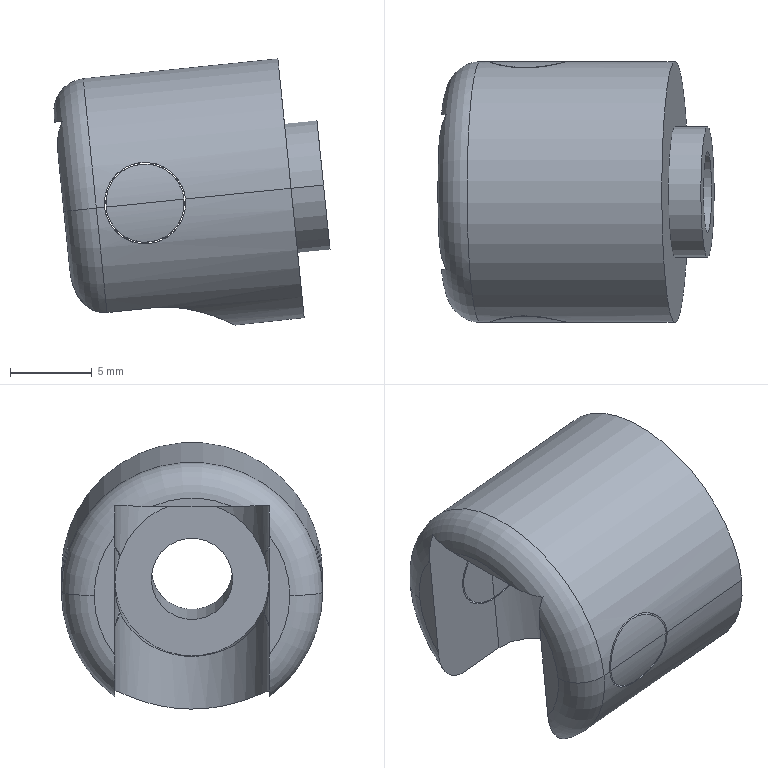Component | SolidWorks | C1-1_C1-1 | 3 solids | 42 faces | box 16.94 x 16 x 16.35 mm | volume 1605 mm3 | cylinder 28 | plane 11 | torus 3 | commonest cylinder face diameters 9.5 x11 5 x6 16 x5 4.8 x4 8 x2
build123d program:
from build123d import *

# Parameters (mm, degrees)
SKETCH1_R               = 8
BOSS_EXTRUDE1_DEPTH     = 14
SKETCH3_R               = 4
BOSS_EXTRUDE2_DEPTH     = 2
FILLET1_R               = 2
SKETCH4_R               = 4.75
CUT_EXTRUDE1_DEPTH      = 10
CUT_EXTRUDE2_DEPTH      = 5.5
CUT_EXTRUDE2_DEPTH_BACK = 20.596
CUT_EXTRUDE3_DEPTH      = 20.596
CUT_EXTRUDE3_DEPTH_BACK = 20.596
SKETCH6_R               = 2.5
SKETCH6_R_2             = 2.4
SKETCH7_R               = 2.5
CUT_EXTRUDE4_DEPTH      = 10


with BuildPart() as part:
    # Sketch1 → Boss-Extrude1 (new body)
    with BuildSketch(Plane.XY):
        Circle(SKETCH1_R)
    extrude(amount=BOSS_EXTRUDE1_DEPTH)

    # Sketch3 → Boss-Extrude2 (add)
    with BuildSketch(Plane.XY.offset(14)):
        Circle(SKETCH3_R)
    extrude(amount=BOSS_EXTRUDE2_DEPTH)

    # Fillet1
    fillet1_edges = [part.edges().sort_by_distance(p)[0] for p in [
        (-8, 0, 0),
    ]]
    fillet(fillet1_edges, radius=FILLET1_R)

    # Sketch4 → Cut-Extrude1 (cut)
    with BuildSketch(Plane(origin=(0, 0, 0), x_dir=(-1, 0, 0), z_dir=(0, 0, -1))):
        Circle(SKETCH4_R)
    extrude(amount=-CUT_EXTRUDE1_DEPTH, mode=Mode.SUBTRACT)

    # Sketch5 → Cut-Extrude2 (cut, two sides: drawn at the far end of the back side and taken through both)
    with BuildSketch(Plane(origin=(0, 0, 0), x_dir=(1, 0, 0), z_dir=(0, 1, 0)).offset(-CUT_EXTRUDE2_DEPTH_BACK)):
        with BuildLine():
            Line((4.75, 5), (4.75, -5))
            ThreePointArc((4.75, -5), (0, -9.75), (-4.75, -5))
            Line((-4.75, -5), (-4.75, 5))
            ThreePointArc((-4.75, 5), (0, 9.75), (4.75, 5))
        make_face()
    extrude(amount=CUT_EXTRUDE2_DEPTH + CUT_EXTRUDE2_DEPTH_BACK, mode=Mode.SUBTRACT)

    # Sketch6 → Cut-Extrude3 (cut, two sides: drawn at the far end of the back side and taken through both)
    with BuildSketch(Plane(origin=(0, 0, 0), x_dir=(0, 0, -1), z_dir=(1, 0, 0)).offset(-CUT_EXTRUDE3_DEPTH_BACK)):
        with Locations((-5, 0)):
            Circle(SKETCH6_R)
        with Locations((-5, 0)):
            Circle(SKETCH6_R_2, mode=Mode.SUBTRACT)
    extrude(amount=CUT_EXTRUDE3_DEPTH + CUT_EXTRUDE3_DEPTH_BACK, mode=Mode.SUBTRACT)


with BuildPart() as cut_extrude3_piece_1:
    # of the separate pieces the step leaves, piece 1, a body of its own (cut_extrude3_pieces)
    add(part.part.solids().sort_by_distance((8, 0, 2))[0])

    # Sketch7 → Cut-Extrude4 (cut)
    with BuildSketch(Plane.XY.offset(16)):
        Circle(SKETCH7_R)
    extrude(amount=-CUT_EXTRUDE4_DEPTH, mode=Mode.SUBTRACT)


with BuildPart() as cut_extrude3_piece_2:
    # of the separate pieces the step leaves, piece 2, a body of its own (cut_extrude3_pieces)
    add(part.part.solids().sort_by_distance((-8, 0, 2.6))[0])


with BuildPart() as cut_extrude3_piece_3:
    # of the separate pieces the step leaves, piece 3, a body of its own (cut_extrude3_pieces)
    add(part.part.solids().sort_by_distance((8, 0, 2.6))[0])


solid = Compound([cut_extrude3_piece_1.part, cut_extrude3_piece_2.part, cut_extrude3_piece_3.part])

# Placed as in the assembly
solid = solid.moved(Location((-282.86, -113.128, 589.605), (0.004478, 84.192, 89.995)))